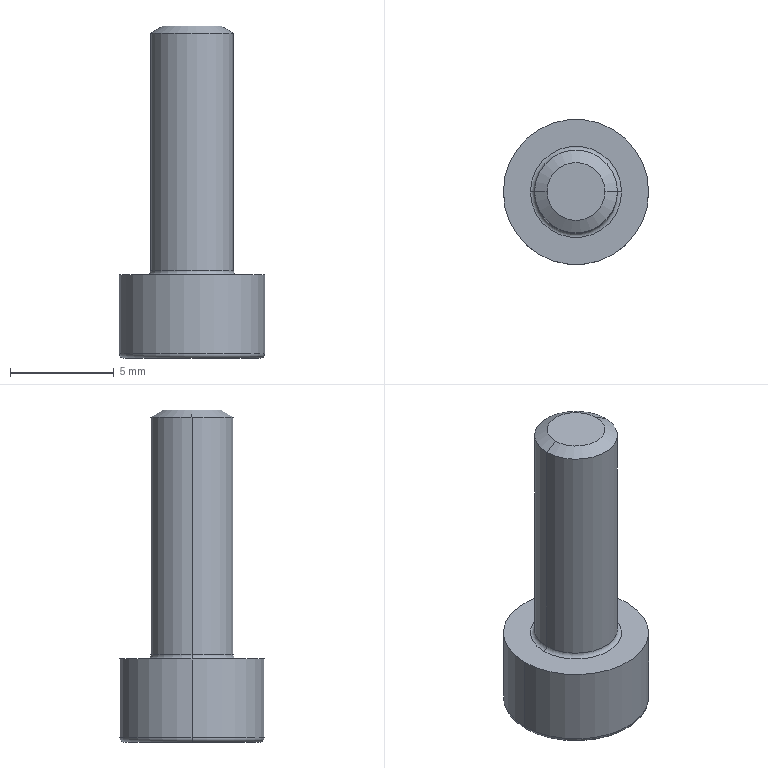Component | SolidWorks | GB_T_70.1-2008[SocketHeadCapScrew_M4_20]-1 | 1 solid | 20 faces | box 7 x 7 x 16 mm | volume 288 mm3 | plane 10 | torus 4 | cylinder 4 | cone 2 | commonest cylinder face diameters 7 x2 4 x2
STEP:
#1=COLOUR_RGB('',0.7922,0.8196,0.9333);
#2=FILL_AREA_STYLE_COLOUR('',#1);
#3=FILL_AREA_STYLE('',(#2));
#4=SURFACE_STYLE_FILL_AREA(#3);
#5=SURFACE_SIDE_STYLE('',(#4));
#6=SURFACE_STYLE_USAGE(.BOTH.,#5);
#7=PRESENTATION_STYLE_ASSIGNMENT((#6));
#8=CARTESIAN_POINT('',(2.211,2.901,-1.669));
#9=VERTEX_POINT('',#8);
#10=CARTESIAN_POINT('',(2.321,2.901,-1.669));
#11=VERTEX_POINT('',#10);
#12=CARTESIAN_POINT('',(2.266,2.901,-1.669));
#13=DIRECTION('',(-0.,-0.,-1.));
#14=DIRECTION('',(-1.,0.,0.));
#15=AXIS2_PLACEMENT_3D('',#12,#13,#14);
#16=CIRCLE('',#15,0.05487);
#17=EDGE_CURVE('',#9,#11,#16,.T.);
#18=ORIENTED_EDGE('',*,*,#17,.T.);
#19=CARTESIAN_POINT('',(2.344,2.901,-1.683));
#20=VERTEX_POINT('',#19);
#21=CARTESIAN_POINT('',(2.344,2.901,-1.683));
#22=DIRECTION('',(0.866,0.,-0.5));
#23=VECTOR('',#22,39.37);
#24=LINE('',#21,#23);
#25=EDGE_CURVE('',#11,#20,#24,.T.);
#26=ORIENTED_EDGE('',*,*,#25,.T.);
#27=CARTESIAN_POINT('',(2.187,2.901,-1.683));
#28=VERTEX_POINT('',#27);
#29=CARTESIAN_POINT('',(2.266,2.901,-1.683));
#30=DIRECTION('',(-0.,-0.,-1.));
#31=DIRECTION('',(-1.,0.,0.));
#32=AXIS2_PLACEMENT_3D('',#29,#30,#31);
#33=CIRCLE('',#32,0.07874);
#34=EDGE_CURVE('',#28,#20,#33,.T.);
#35=ORIENTED_EDGE('',*,*,#34,.F.);
#36=CARTESIAN_POINT('',(2.187,2.901,-1.683));
#37=DIRECTION('',(-0.866,-0.,-0.5));
#38=VECTOR('',#37,39.37);
#39=LINE('',#36,#38);
#40=EDGE_CURVE('',#9,#28,#39,.T.);
#41=ORIENTED_EDGE('',*,*,#40,.F.);
#42=EDGE_LOOP('',(#18,#26,#35,#41));
#43=FACE_OUTER_BOUND('',#42,.T.);
#44=CARTESIAN_POINT('',(2.266,2.901,-1.683));
#45=DIRECTION('',(-0.,-0.,-1.));
#46=DIRECTION('',(-1.,0.,0.));
#47=AXIS2_PLACEMENT_3D('',#44,#45,#46);
#48=CONICAL_SURFACE('',#47,0.07874,1.047);
#49=ADVANCED_FACE('',(#43),#48,.T.);
#50=CARTESIAN_POINT('',(2.403,2.901,-2.291));
#51=VERTEX_POINT('',#50);
#52=CARTESIAN_POINT('',(2.128,2.901,-2.291));
#53=VERTEX_POINT('',#52);
#54=CARTESIAN_POINT('',(2.266,2.901,-2.291));
#55=DIRECTION('',(0.,0.,1.));
#56=DIRECTION('',(-1.,0.,0.));
#57=AXIS2_PLACEMENT_3D('',#54,#55,#56);
#58=CIRCLE('',#57,0.1378);
#59=EDGE_CURVE('',#51,#53,#58,.T.);
#60=ORIENTED_EDGE('',*,*,#59,.F.);
#61=CARTESIAN_POINT('',(2.396,2.901,-2.299));
#62=VERTEX_POINT('',#61);
#63=CARTESIAN_POINT('',(2.396,2.901,-2.291));
#64=DIRECTION('',(-0.,1.,-0.));
#65=DIRECTION('',(-1.,0.,0.));
#66=AXIS2_PLACEMENT_3D('',#63,#64,#65);
#67=CIRCLE('',#66,0.007874);
#68=EDGE_CURVE('',#51,#62,#67,.T.);
#69=ORIENTED_EDGE('',*,*,#68,.T.);
#70=CARTESIAN_POINT('',(2.136,2.901,-2.299));
#71=VERTEX_POINT('',#70);
#72=CARTESIAN_POINT('',(2.266,2.901,-2.299));
#73=DIRECTION('',(-0.,-0.,-1.));
#74=DIRECTION('',(-1.,0.,0.));
#75=AXIS2_PLACEMENT_3D('',#72,#73,#74);
#76=CIRCLE('',#75,0.1299);
#77=EDGE_CURVE('',#71,#62,#76,.T.);
#78=ORIENTED_EDGE('',*,*,#77,.F.);
#79=CARTESIAN_POINT('',(2.136,2.901,-2.291));
#80=DIRECTION('',(0.,-1.,0.));
#81=DIRECTION('',(0.,0.,-1.));
#82=AXIS2_PLACEMENT_3D('',#79,#80,#81);
#83=CIRCLE('',#82,0.007874);
#84=EDGE_CURVE('',#53,#71,#83,.T.);
#85=ORIENTED_EDGE('',*,*,#84,.F.);
#86=EDGE_LOOP('',(#60,#69,#78,#85));
#87=FACE_OUTER_BOUND('',#86,.T.);
#88=CARTESIAN_POINT('',(2.266,2.901,-2.291));
#89=DIRECTION('',(-0.,-0.,-1.));
#90=DIRECTION('',(-1.,0.,0.));
#91=AXIS2_PLACEMENT_3D('',#88,#89,#90);
#92=TOROIDAL_SURFACE('',#91,0.1299,0.007874);
#93=ADVANCED_FACE('',(#87),#92,.T.);
#94=CARTESIAN_POINT('',(2.187,2.901,-2.134));
#95=VERTEX_POINT('',#94);
#96=CARTESIAN_POINT('',(2.344,2.901,-2.134));
#97=VERTEX_POINT('',#96);
#98=CARTESIAN_POINT('',(2.266,2.901,-2.134));
#99=DIRECTION('',(0.,0.,1.));
#100=DIRECTION('',(1.,0.,0.));
#101=AXIS2_PLACEMENT_3D('',#98,#99,#100);
#102=CIRCLE('',#101,0.07874);
#103=EDGE_CURVE('',#95,#97,#102,.T.);
#104=ORIENTED_EDGE('',*,*,#103,.F.);
#105=CARTESIAN_POINT('',(2.179,2.901,-2.142));
#106=VERTEX_POINT('',#105);
#107=CARTESIAN_POINT('',(2.179,2.901,-2.134));
#108=DIRECTION('',(-0.,1.,-0.));
#109=DIRECTION('',(0.,0.,1.));
#110=AXIS2_PLACEMENT_3D('',#107,#108,#109);
#111=CIRCLE('',#110,0.007874);
#112=EDGE_CURVE('',#95,#106,#111,.T.);
#113=ORIENTED_EDGE('',*,*,#112,.T.);
#114=CARTESIAN_POINT('',(2.352,2.901,-2.142));
#115=VERTEX_POINT('',#114);
#116=CARTESIAN_POINT('',(2.266,2.901,-2.142));
#117=DIRECTION('',(0.,0.,1.));
#118=DIRECTION('',(1.,0.,0.));
#119=AXIS2_PLACEMENT_3D('',#116,#117,#118);
#120=CIRCLE('',#119,0.08661);
#121=EDGE_CURVE('',#106,#115,#120,.T.);
#122=ORIENTED_EDGE('',*,*,#121,.T.);
#123=CARTESIAN_POINT('',(2.352,2.901,-2.134));
#124=DIRECTION('',(0.,-1.,0.));
#125=DIRECTION('',(0.,0.,-1.));
#126=AXIS2_PLACEMENT_3D('',#123,#124,#125);
#127=CIRCLE('',#126,0.007874);
#128=EDGE_CURVE('',#97,#115,#127,.T.);
#129=ORIENTED_EDGE('',*,*,#128,.F.);
#130=EDGE_LOOP('',(#104,#113,#122,#129));
#131=FACE_OUTER_BOUND('',#130,.T.);
#132=CARTESIAN_POINT('',(2.266,2.901,-2.134));
#133=DIRECTION('',(0.,0.,1.));
#134=DIRECTION('',(1.,-0.,-0.));
#135=AXIS2_PLACEMENT_3D('',#132,#133,#134);
#136=TOROIDAL_SURFACE('',#135,0.08661,0.007874);
#137=ADVANCED_FACE('',(#131),#136,.F.);
#138=ORIENTED_EDGE('',*,*,#59,.T.);
#139=CARTESIAN_POINT('',(2.128,2.901,-2.142));
#140=VERTEX_POINT('',#139);
#141=CARTESIAN_POINT('',(2.128,2.901,-2.299));
#142=DIRECTION('',(0.,0.,1.));
#143=VECTOR('',#142,39.37);
#144=LINE('',#141,#143);
#145=EDGE_CURVE('',#53,#140,#144,.T.);
#146=ORIENTED_EDGE('',*,*,#145,.T.);
#147=CARTESIAN_POINT('',(2.403,2.901,-2.142));
#148=VERTEX_POINT('',#147);
#149=CARTESIAN_POINT('',(2.266,2.901,-2.142));
#150=DIRECTION('',(0.,0.,1.));
#151=DIRECTION('',(1.,0.,0.));
#152=AXIS2_PLACEMENT_3D('',#149,#150,#151);
#153=CIRCLE('',#152,0.1378);
#154=EDGE_CURVE('',#148,#140,#153,.T.);
#155=ORIENTED_EDGE('',*,*,#154,.F.);
#156=CARTESIAN_POINT('',(2.403,2.901,-2.299));
#157=DIRECTION('',(0.,0.,1.));
#158=VECTOR('',#157,39.37);
#159=LINE('',#156,#158);
#160=EDGE_CURVE('',#51,#148,#159,.T.);
#161=ORIENTED_EDGE('',*,*,#160,.F.);
#162=EDGE_LOOP('',(#138,#146,#155,#161));
#163=FACE_OUTER_BOUND('',#162,.T.);
#164=CARTESIAN_POINT('',(2.266,2.901,-2.299));
#165=DIRECTION('',(0.,0.,1.));
#166=DIRECTION('',(1.,0.,0.));
#167=AXIS2_PLACEMENT_3D('',#164,#165,#166);
#168=CYLINDRICAL_SURFACE('',#167,0.1378);
#169=ADVANCED_FACE('',(#163),#168,.T.);
#170=CARTESIAN_POINT('',(2.266,2.901,-2.134));
#171=DIRECTION('',(0.,0.,1.));
#172=DIRECTION('',(1.,0.,0.));
#173=AXIS2_PLACEMENT_3D('',#170,#171,#172);
#174=CIRCLE('',#173,0.07874);
#175=EDGE_CURVE('',#97,#95,#174,.T.);
#176=ORIENTED_EDGE('',*,*,#175,.T.);
#177=CARTESIAN_POINT('',(2.187,2.901,-2.299));
#178=DIRECTION('',(0.,0.,1.));
#179=VECTOR('',#178,39.37);
#180=LINE('',#177,#179);
#181=EDGE_CURVE('',#95,#28,#180,.T.);
#182=ORIENTED_EDGE('',*,*,#181,.T.);
#183=ORIENTED_EDGE('',*,*,#34,.T.);
#184=CARTESIAN_POINT('',(2.344,2.901,-2.299));
#185=DIRECTION('',(0.,0.,1.));
#186=VECTOR('',#185,39.37);
#187=LINE('',#184,#186);
#188=EDGE_CURVE('',#97,#20,#187,.T.);
#189=ORIENTED_EDGE('',*,*,#188,.F.);
#190=EDGE_LOOP('',(#176,#182,#183,#189));
#191=FACE_OUTER_BOUND('',#190,.T.);
#192=CARTESIAN_POINT('',(2.266,2.901,-2.299));
#193=DIRECTION('',(0.,0.,1.));
#194=DIRECTION('',(1.,0.,0.));
#195=AXIS2_PLACEMENT_3D('',#192,#193,#194);
#196=CYLINDRICAL_SURFACE('',#195,0.07874);
#197=ADVANCED_FACE('',(#191),#196,.T.);
#198=ORIENTED_EDGE('',*,*,#181,.F.);
#199=ORIENTED_EDGE('',*,*,#103,.T.);
#200=ORIENTED_EDGE('',*,*,#188,.T.);
#201=CARTESIAN_POINT('',(2.266,2.901,-1.683));
#202=DIRECTION('',(-0.,-0.,-1.));
#203=DIRECTION('',(-1.,0.,0.));
#204=AXIS2_PLACEMENT_3D('',#201,#202,#203);
#205=CIRCLE('',#204,0.07874);
#206=EDGE_CURVE('',#20,#28,#205,.T.);
#207=ORIENTED_EDGE('',*,*,#206,.T.);
#208=EDGE_LOOP('',(#198,#199,#200,#207));
#209=FACE_OUTER_BOUND('',#208,.T.);
#210=CARTESIAN_POINT('',(2.266,2.901,-2.299));
#211=DIRECTION('',(0.,0.,1.));
#212=DIRECTION('',(1.,0.,0.));
#213=AXIS2_PLACEMENT_3D('',#210,#211,#212);
#214=CYLINDRICAL_SURFACE('',#213,0.07874);
#215=ADVANCED_FACE('',(#209),#214,.T.);
#216=ORIENTED_EDGE('',*,*,#77,.T.);
#217=CARTESIAN_POINT('',(2.266,2.901,-2.299));
#218=DIRECTION('',(-0.,-0.,-1.));
#219=DIRECTION('',(-1.,0.,0.));
#220=AXIS2_PLACEMENT_3D('',#217,#218,#219);
#221=CIRCLE('',#220,0.1299);
#222=EDGE_CURVE('',#62,#71,#221,.T.);
#223=ORIENTED_EDGE('',*,*,#222,.T.);
#224=EDGE_LOOP('',(#216,#223));
#225=FACE_OUTER_BOUND('',#224,.T.);
#226=CARTESIAN_POINT('',(2.266,2.834,-2.299));
#227=VERTEX_POINT('',#226);
#228=CARTESIAN_POINT('',(2.207,2.868,-2.299));
#229=VERTEX_POINT('',#228);
#230=CARTESIAN_POINT('',(2.266,2.834,-2.299));
#231=DIRECTION('',(-0.866,0.5,-0.));
#232=VECTOR('',#231,39.37);
#233=LINE('',#230,#232);
#234=EDGE_CURVE('',#227,#229,#233,.T.);
#235=ORIENTED_EDGE('',*,*,#234,.F.);
#236=CARTESIAN_POINT('',(2.324,2.868,-2.299));
#237=VERTEX_POINT('',#236);
#238=CARTESIAN_POINT('',(2.324,2.868,-2.299));
#239=DIRECTION('',(-0.866,-0.5,0.));
#240=VECTOR('',#239,39.37);
#241=LINE('',#238,#240);
#242=EDGE_CURVE('',#237,#227,#241,.T.);
#243=ORIENTED_EDGE('',*,*,#242,.F.);
#244=CARTESIAN_POINT('',(2.324,2.935,-2.299));
#245=VERTEX_POINT('',#244);
#246=CARTESIAN_POINT('',(2.324,2.935,-2.299));
#247=DIRECTION('',(0.,-1.,0.));
#248=VECTOR('',#247,39.37);
#249=LINE('',#246,#248);
#250=EDGE_CURVE('',#245,#237,#249,.T.);
#251=ORIENTED_EDGE('',*,*,#250,.F.);
#252=CARTESIAN_POINT('',(2.266,2.969,-2.299));
#253=VERTEX_POINT('',#252);
#254=CARTESIAN_POINT('',(2.266,2.969,-2.299));
#255=DIRECTION('',(0.866,-0.5,0.));
#256=VECTOR('',#255,39.37);
#257=LINE('',#254,#256);
#258=EDGE_CURVE('',#253,#245,#257,.T.);
#259=ORIENTED_EDGE('',*,*,#258,.F.);
#260=CARTESIAN_POINT('',(2.207,2.935,-2.299));
#261=VERTEX_POINT('',#260);
#262=CARTESIAN_POINT('',(2.207,2.935,-2.299));
#263=DIRECTION('',(0.866,0.5,-0.));
#264=VECTOR('',#263,39.37);
#265=LINE('',#262,#264);
#266=EDGE_CURVE('',#261,#253,#265,.T.);
#267=ORIENTED_EDGE('',*,*,#266,.F.);
#268=CARTESIAN_POINT('',(2.207,2.868,-2.299));
#269=DIRECTION('',(-0.,1.,-0.));
#270=VECTOR('',#269,39.37);
#271=LINE('',#268,#270);
#272=EDGE_CURVE('',#229,#261,#271,.T.);
#273=ORIENTED_EDGE('',*,*,#272,.F.);
#274=EDGE_LOOP('',(#235,#243,#251,#259,#267,#273));
#275=FACE_BOUND('',#274,.T.);
#276=CARTESIAN_POINT('',(2.266,2.901,-2.299));
#277=DIRECTION('',(-0.,-0.,-1.));
#278=DIRECTION('',(-1.,-0.,0.));
#279=AXIS2_PLACEMENT_3D('',#276,#277,#278);
#280=PLANE('',#279);
#281=ADVANCED_FACE('',(#225,#275),#280,.T.);
#282=ORIENTED_EDGE('',*,*,#145,.F.);
#283=CARTESIAN_POINT('',(2.266,2.901,-2.291));
#284=DIRECTION('',(0.,0.,1.));
#285=DIRECTION('',(-1.,0.,0.));
#286=AXIS2_PLACEMENT_3D('',#283,#284,#285);
#287=CIRCLE('',#286,0.1378);
#288=EDGE_CURVE('',#53,#51,#287,.T.);
#289=ORIENTED_EDGE('',*,*,#288,.T.);
#290=ORIENTED_EDGE('',*,*,#160,.T.);
#291=CARTESIAN_POINT('',(2.266,2.901,-2.142));
#292=DIRECTION('',(0.,0.,1.));
#293=DIRECTION('',(1.,0.,0.));
#294=AXIS2_PLACEMENT_3D('',#291,#292,#293);
#295=CIRCLE('',#294,0.1378);
#296=EDGE_CURVE('',#140,#148,#295,.T.);
#297=ORIENTED_EDGE('',*,*,#296,.F.);
#298=EDGE_LOOP('',(#282,#289,#290,#297));
#299=FACE_OUTER_BOUND('',#298,.T.);
#300=CARTESIAN_POINT('',(2.266,2.901,-2.299));
#301=DIRECTION('',(0.,0.,1.));
#302=DIRECTION('',(1.,0.,0.));
#303=AXIS2_PLACEMENT_3D('',#300,#301,#302);
#304=CYLINDRICAL_SURFACE('',#303,0.1378);
#305=ADVANCED_FACE('',(#299),#304,.T.);
#306=ORIENTED_EDGE('',*,*,#154,.T.);
#307=ORIENTED_EDGE('',*,*,#296,.T.);
#308=EDGE_LOOP('',(#306,#307));
#309=FACE_OUTER_BOUND('',#308,.T.);
#310=CARTESIAN_POINT('',(2.266,2.901,-2.142));
#311=DIRECTION('',(0.,0.,1.));
#312=DIRECTION('',(1.,0.,0.));
#313=AXIS2_PLACEMENT_3D('',#310,#311,#312);
#314=CIRCLE('',#313,0.08661);
#315=EDGE_CURVE('',#115,#106,#314,.T.);
#316=ORIENTED_EDGE('',*,*,#315,.F.);
#317=ORIENTED_EDGE('',*,*,#121,.F.);
#318=EDGE_LOOP('',(#316,#317));
#319=FACE_BOUND('',#318,.T.);
#320=CARTESIAN_POINT('',(2.266,3.039,-2.142));
#321=DIRECTION('',(0.,0.,1.));
#322=DIRECTION('',(1.,0.,-0.));
#323=AXIS2_PLACEMENT_3D('',#320,#321,#322);
#324=PLANE('',#323);
#325=ADVANCED_FACE('',(#309,#319),#324,.T.);
#326=ORIENTED_EDGE('',*,*,#112,.F.);
#327=ORIENTED_EDGE('',*,*,#175,.F.);
#328=ORIENTED_EDGE('',*,*,#128,.T.);
#329=ORIENTED_EDGE('',*,*,#315,.T.);
#330=EDGE_LOOP('',(#326,#327,#328,#329));
#331=FACE_OUTER_BOUND('',#330,.T.);
#332=CARTESIAN_POINT('',(2.266,2.901,-2.134));
#333=DIRECTION('',(0.,0.,1.));
#334=DIRECTION('',(1.,-0.,-0.));
#335=AXIS2_PLACEMENT_3D('',#332,#333,#334);
#336=TOROIDAL_SURFACE('',#335,0.08661,0.007874);
#337=ADVANCED_FACE('',(#331),#336,.F.);
#338=ORIENTED_EDGE('',*,*,#234,.T.);
#339=CARTESIAN_POINT('',(2.207,2.868,-2.22));
#340=VERTEX_POINT('',#339);
#341=CARTESIAN_POINT('',(2.207,2.868,-2.22));
#342=DIRECTION('',(-0.,-0.,-1.));
#343=VECTOR('',#342,39.37);
#344=LINE('',#341,#343);
#345=EDGE_CURVE('',#340,#229,#344,.T.);
#346=ORIENTED_EDGE('',*,*,#345,.F.);
#347=CARTESIAN_POINT('',(2.266,2.834,-2.22));
#348=VERTEX_POINT('',#347);
#349=CARTESIAN_POINT('',(2.266,2.834,-2.22));
#350=DIRECTION('',(-0.866,0.5,-0.));
#351=VECTOR('',#350,39.37);
#352=LINE('',#349,#351);
#353=EDGE_CURVE('',#348,#340,#352,.T.);
#354=ORIENTED_EDGE('',*,*,#353,.F.);
#355=CARTESIAN_POINT('',(2.266,2.834,-2.22));
#356=DIRECTION('',(-0.,-0.,-1.));
#357=VECTOR('',#356,39.37);
#358=LINE('',#355,#357);
#359=EDGE_CURVE('',#348,#227,#358,.T.);
#360=ORIENTED_EDGE('',*,*,#359,.T.);
#361=EDGE_LOOP('',(#338,#346,#354,#360));
#362=FACE_OUTER_BOUND('',#361,.T.);
#363=CARTESIAN_POINT('',(2.266,2.834,-2.22));
#364=DIRECTION('',(-0.5,-0.866,0.));
#365=DIRECTION('',(0.866,-0.5,0.));
#366=AXIS2_PLACEMENT_3D('',#363,#364,#365);
#367=PLANE('',#366);
#368=ADVANCED_FACE('',(#362),#367,.F.);
#369=ORIENTED_EDGE('',*,*,#242,.T.);
#370=ORIENTED_EDGE('',*,*,#359,.F.);
#371=CARTESIAN_POINT('',(2.324,2.868,-2.22));
#372=VERTEX_POINT('',#371);
#373=CARTESIAN_POINT('',(2.324,2.868,-2.22));
#374=DIRECTION('',(-0.866,-0.5,0.));
#375=VECTOR('',#374,39.37);
#376=LINE('',#373,#375);
#377=EDGE_CURVE('',#372,#348,#376,.T.);
#378=ORIENTED_EDGE('',*,*,#377,.F.);
#379=CARTESIAN_POINT('',(2.324,2.868,-2.22));
#380=DIRECTION('',(-0.,-0.,-1.));
#381=VECTOR('',#380,39.37);
#382=LINE('',#379,#381);
#383=EDGE_CURVE('',#372,#237,#382,.T.);
#384=ORIENTED_EDGE('',*,*,#383,.T.);
#385=EDGE_LOOP('',(#369,#370,#378,#384));
#386=FACE_OUTER_BOUND('',#385,.T.);
#387=CARTESIAN_POINT('',(2.324,2.868,-2.22));
#388=DIRECTION('',(0.5,-0.866,0.));
#389=DIRECTION('',(0.866,0.5,-0.));
#390=AXIS2_PLACEMENT_3D('',#387,#388,#389);
#391=PLANE('',#390);
#392=ADVANCED_FACE('',(#386),#391,.F.);
#393=ORIENTED_EDGE('',*,*,#250,.T.);
#394=ORIENTED_EDGE('',*,*,#383,.F.);
#395=CARTESIAN_POINT('',(2.324,2.935,-2.22));
#396=VERTEX_POINT('',#395);
#397=CARTESIAN_POINT('',(2.324,2.935,-2.22));
#398=DIRECTION('',(0.,-1.,0.));
#399=VECTOR('',#398,39.37);
#400=LINE('',#397,#399);
#401=EDGE_CURVE('',#396,#372,#400,.T.);
#402=ORIENTED_EDGE('',*,*,#401,.F.);
#403=CARTESIAN_POINT('',(2.324,2.935,-2.22));
#404=DIRECTION('',(-0.,-0.,-1.));
#405=VECTOR('',#404,39.37);
#406=LINE('',#403,#405);
#407=EDGE_CURVE('',#396,#245,#406,.T.);
#408=ORIENTED_EDGE('',*,*,#407,.T.);
#409=EDGE_LOOP('',(#393,#394,#402,#408));
#410=FACE_OUTER_BOUND('',#409,.T.);
#411=CARTESIAN_POINT('',(2.324,2.935,-2.22));
#412=DIRECTION('',(1.,0.,-0.));
#413=DIRECTION('',(-0.,1.,-0.));
#414=AXIS2_PLACEMENT_3D('',#411,#412,#413);
#415=PLANE('',#414);
#416=ADVANCED_FACE('',(#410),#415,.F.);
#417=ORIENTED_EDGE('',*,*,#258,.T.);
#418=ORIENTED_EDGE('',*,*,#407,.F.);
#419=CARTESIAN_POINT('',(2.266,2.969,-2.22));
#420=VERTEX_POINT('',#419);
#421=CARTESIAN_POINT('',(2.266,2.969,-2.22));
#422=DIRECTION('',(0.866,-0.5,0.));
#423=VECTOR('',#422,39.37);
#424=LINE('',#421,#423);
#425=EDGE_CURVE('',#420,#396,#424,.T.);
#426=ORIENTED_EDGE('',*,*,#425,.F.);
#427=CARTESIAN_POINT('',(2.266,2.969,-2.22));
#428=DIRECTION('',(-0.,-0.,-1.));
#429=VECTOR('',#428,39.37);
#430=LINE('',#427,#429);
#431=EDGE_CURVE('',#420,#253,#430,.T.);
#432=ORIENTED_EDGE('',*,*,#431,.T.);
#433=EDGE_LOOP('',(#417,#418,#426,#432));
#434=FACE_OUTER_BOUND('',#433,.T.);
#435=CARTESIAN_POINT('',(2.266,2.969,-2.22));
#436=DIRECTION('',(0.5,0.866,-0.));
#437=DIRECTION('',(-0.866,0.5,-0.));
#438=AXIS2_PLACEMENT_3D('',#435,#436,#437);
#439=PLANE('',#438);
#440=ADVANCED_FACE('',(#434),#439,.F.);
#441=ORIENTED_EDGE('',*,*,#266,.T.);
#442=ORIENTED_EDGE('',*,*,#431,.F.);
#443=CARTESIAN_POINT('',(2.207,2.935,-2.22));
#444=VERTEX_POINT('',#443);
#445=CARTESIAN_POINT('',(2.207,2.935,-2.22));
#446=DIRECTION('',(0.866,0.5,-0.));
#447=VECTOR('',#446,39.37);
#448=LINE('',#445,#447);
#449=EDGE_CURVE('',#444,#420,#448,.T.);
#450=ORIENTED_EDGE('',*,*,#449,.F.);
#451=CARTESIAN_POINT('',(2.207,2.935,-2.22));
#452=DIRECTION('',(-0.,-0.,-1.));
#453=VECTOR('',#452,39.37);
#454=LINE('',#451,#453);
#455=EDGE_CURVE('',#444,#261,#454,.T.);
#456=ORIENTED_EDGE('',*,*,#455,.T.);
#457=EDGE_LOOP('',(#441,#442,#450,#456));
#458=FACE_OUTER_BOUND('',#457,.T.);
#459=CARTESIAN_POINT('',(2.207,2.935,-2.22));
#460=DIRECTION('',(-0.5,0.866,-0.));
#461=DIRECTION('',(-0.866,-0.5,0.));
#462=AXIS2_PLACEMENT_3D('',#459,#460,#461);
#463=PLANE('',#462);
#464=ADVANCED_FACE('',(#458),#463,.F.);
#465=ORIENTED_EDGE('',*,*,#272,.T.);
#466=ORIENTED_EDGE('',*,*,#455,.F.);
#467=CARTESIAN_POINT('',(2.207,2.868,-2.22));
#468=DIRECTION('',(-0.,1.,-0.));
#469=VECTOR('',#468,39.37);
#470=LINE('',#467,#469);
#471=EDGE_CURVE('',#340,#444,#470,.T.);
#472=ORIENTED_EDGE('',*,*,#471,.F.);
#473=ORIENTED_EDGE('',*,*,#345,.T.);
#474=EDGE_LOOP('',(#465,#466,#472,#473));
#475=FACE_OUTER_BOUND('',#474,.T.);
#476=CARTESIAN_POINT('',(2.207,2.868,-2.22));
#477=DIRECTION('',(-1.,-0.,0.));
#478=DIRECTION('',(0.,-1.,0.));
#479=AXIS2_PLACEMENT_3D('',#476,#477,#478);
#480=PLANE('',#479);
#481=ADVANCED_FACE('',(#475),#480,.F.);
#482=ORIENTED_EDGE('',*,*,#353,.T.);
#483=ORIENTED_EDGE('',*,*,#471,.T.);
#484=ORIENTED_EDGE('',*,*,#449,.T.);
#485=ORIENTED_EDGE('',*,*,#425,.T.);
#486=ORIENTED_EDGE('',*,*,#401,.T.);
#487=ORIENTED_EDGE('',*,*,#377,.T.);
#488=EDGE_LOOP('',(#482,#483,#484,#485,#486,#487));
#489=FACE_OUTER_BOUND('',#488,.T.);
#490=CARTESIAN_POINT('',(2.207,2.868,-2.22));
#491=DIRECTION('',(-0.,-0.,-1.));
#492=DIRECTION('',(-1.,-0.,0.));
#493=AXIS2_PLACEMENT_3D('',#490,#491,#492);
#494=PLANE('',#493);
#495=ADVANCED_FACE('',(#489),#494,.T.);
#496=ORIENTED_EDGE('',*,*,#68,.F.);
#497=ORIENTED_EDGE('',*,*,#288,.F.);
#498=ORIENTED_EDGE('',*,*,#84,.T.);
#499=ORIENTED_EDGE('',*,*,#222,.F.);
#500=EDGE_LOOP('',(#496,#497,#498,#499));
#501=FACE_OUTER_BOUND('',#500,.T.);
#502=CARTESIAN_POINT('',(2.266,2.901,-2.291));
#503=DIRECTION('',(-0.,-0.,-1.));
#504=DIRECTION('',(-1.,0.,0.));
#505=AXIS2_PLACEMENT_3D('',#502,#503,#504);
#506=TOROIDAL_SURFACE('',#505,0.1299,0.007874);
#507=ADVANCED_FACE('',(#501),#506,.T.);
#508=ORIENTED_EDGE('',*,*,#25,.F.);
#509=CARTESIAN_POINT('',(2.266,2.901,-1.669));
#510=DIRECTION('',(-0.,-0.,-1.));
#511=DIRECTION('',(-1.,0.,0.));
#512=AXIS2_PLACEMENT_3D('',#509,#510,#511);
#513=CIRCLE('',#512,0.05487);
#514=EDGE_CURVE('',#11,#9,#513,.T.);
#515=ORIENTED_EDGE('',*,*,#514,.T.);
#516=ORIENTED_EDGE('',*,*,#40,.T.);
#517=ORIENTED_EDGE('',*,*,#206,.F.);
#518=EDGE_LOOP('',(#508,#515,#516,#517));
#519=FACE_OUTER_BOUND('',#518,.T.);
#520=CARTESIAN_POINT('',(2.266,2.901,-1.683));
#521=DIRECTION('',(-0.,-0.,-1.));
#522=DIRECTION('',(-1.,0.,0.));
#523=AXIS2_PLACEMENT_3D('',#520,#521,#522);
#524=CONICAL_SURFACE('',#523,0.07874,1.047);
#525=ADVANCED_FACE('',(#519),#524,.T.);
#526=ORIENTED_EDGE('',*,*,#17,.F.);
#527=ORIENTED_EDGE('',*,*,#514,.F.);
#528=EDGE_LOOP('',(#526,#527));
#529=FACE_OUTER_BOUND('',#528,.T.);
#530=CARTESIAN_POINT('',(2.266,2.98,-1.669));
#531=DIRECTION('',(0.,0.,1.));
#532=DIRECTION('',(1.,0.,-0.));
#533=AXIS2_PLACEMENT_3D('',#530,#531,#532);
#534=PLANE('',#533);
#535=ADVANCED_FACE('',(#529),#534,.T.);
#536=CLOSED_SHELL('',(#49,#93,#137,#169,#197,#215,#281,#305,#325,#337,#368,#392,#416,#440,#464,#481,#495,#507,#525,#535));
#537=MANIFOLD_SOLID_BREP('',#536);
#538=STYLED_ITEM('',(#7),#537);
#539=PRESENTATION_LAYER_ASSIGNMENT('','',(#538));
#540=CARTESIAN_POINT('',(0.,0.,0.));
#541=DIRECTION('',(0.,0.,1.));
#542=DIRECTION('',(1.,0.,0.));
#543=AXIS2_PLACEMENT_3D('',#540,#541,#542);
#544=(LENGTH_UNIT()NAMED_UNIT(*)SI_UNIT($,.METRE.));
#545=LENGTH_MEASURE_WITH_UNIT(LENGTH_MEASURE(0.0254),#544);
#546=DIMENSIONAL_EXPONENTS(1.,0.,0.,0.,0.,0.,0.);
#547=(CONVERSION_BASED_UNIT('',#545)LENGTH_UNIT()NAMED_UNIT(#546));
#548=UNCERTAINTY_MEASURE_WITH_UNIT(LENGTH_MEASURE(0.00001),#547,'','');
#549=(NAMED_UNIT(*)PLANE_ANGLE_UNIT()SI_UNIT($,.RADIAN.));
#550=(NAMED_UNIT(*)SI_UNIT($,.STERADIAN.)SOLID_ANGLE_UNIT());
#551=(GEOMETRIC_REPRESENTATION_CONTEXT(3)GLOBAL_UNCERTAINTY_ASSIGNED_CONTEXT((#548))GLOBAL_UNIT_ASSIGNED_CONTEXT((#547,#549,#550))REPRESENTATION_CONTEXT('',''));
#552=ADVANCED_BREP_SHAPE_REPRESENTATION('',(#537,#543),#551);
#553=(LENGTH_UNIT()NAMED_UNIT(*)SI_UNIT($,.METRE.));
#554=LENGTH_MEASURE_WITH_UNIT(LENGTH_MEASURE(0.0254),#553);
#555=DIMENSIONAL_EXPONENTS(1.,0.,0.,0.,0.,0.,0.);
#556=(CONVERSION_BASED_UNIT('',#554)LENGTH_UNIT()NAMED_UNIT(#555));
#557=UNCERTAINTY_MEASURE_WITH_UNIT(LENGTH_MEASURE(0.00001),#556,'','');
#558=(NAMED_UNIT(*)PLANE_ANGLE_UNIT()SI_UNIT($,.RADIAN.));
#559=(NAMED_UNIT(*)SI_UNIT($,.STERADIAN.)SOLID_ANGLE_UNIT());
#560=(GEOMETRIC_REPRESENTATION_CONTEXT(3)GLOBAL_UNCERTAINTY_ASSIGNED_CONTEXT((#557))GLOBAL_UNIT_ASSIGNED_CONTEXT((#556,#558,#559))REPRESENTATION_CONTEXT('',''));
#561=MECHANICAL_DESIGN_GEOMETRIC_PRESENTATION_REPRESENTATION('',(#538),#560);